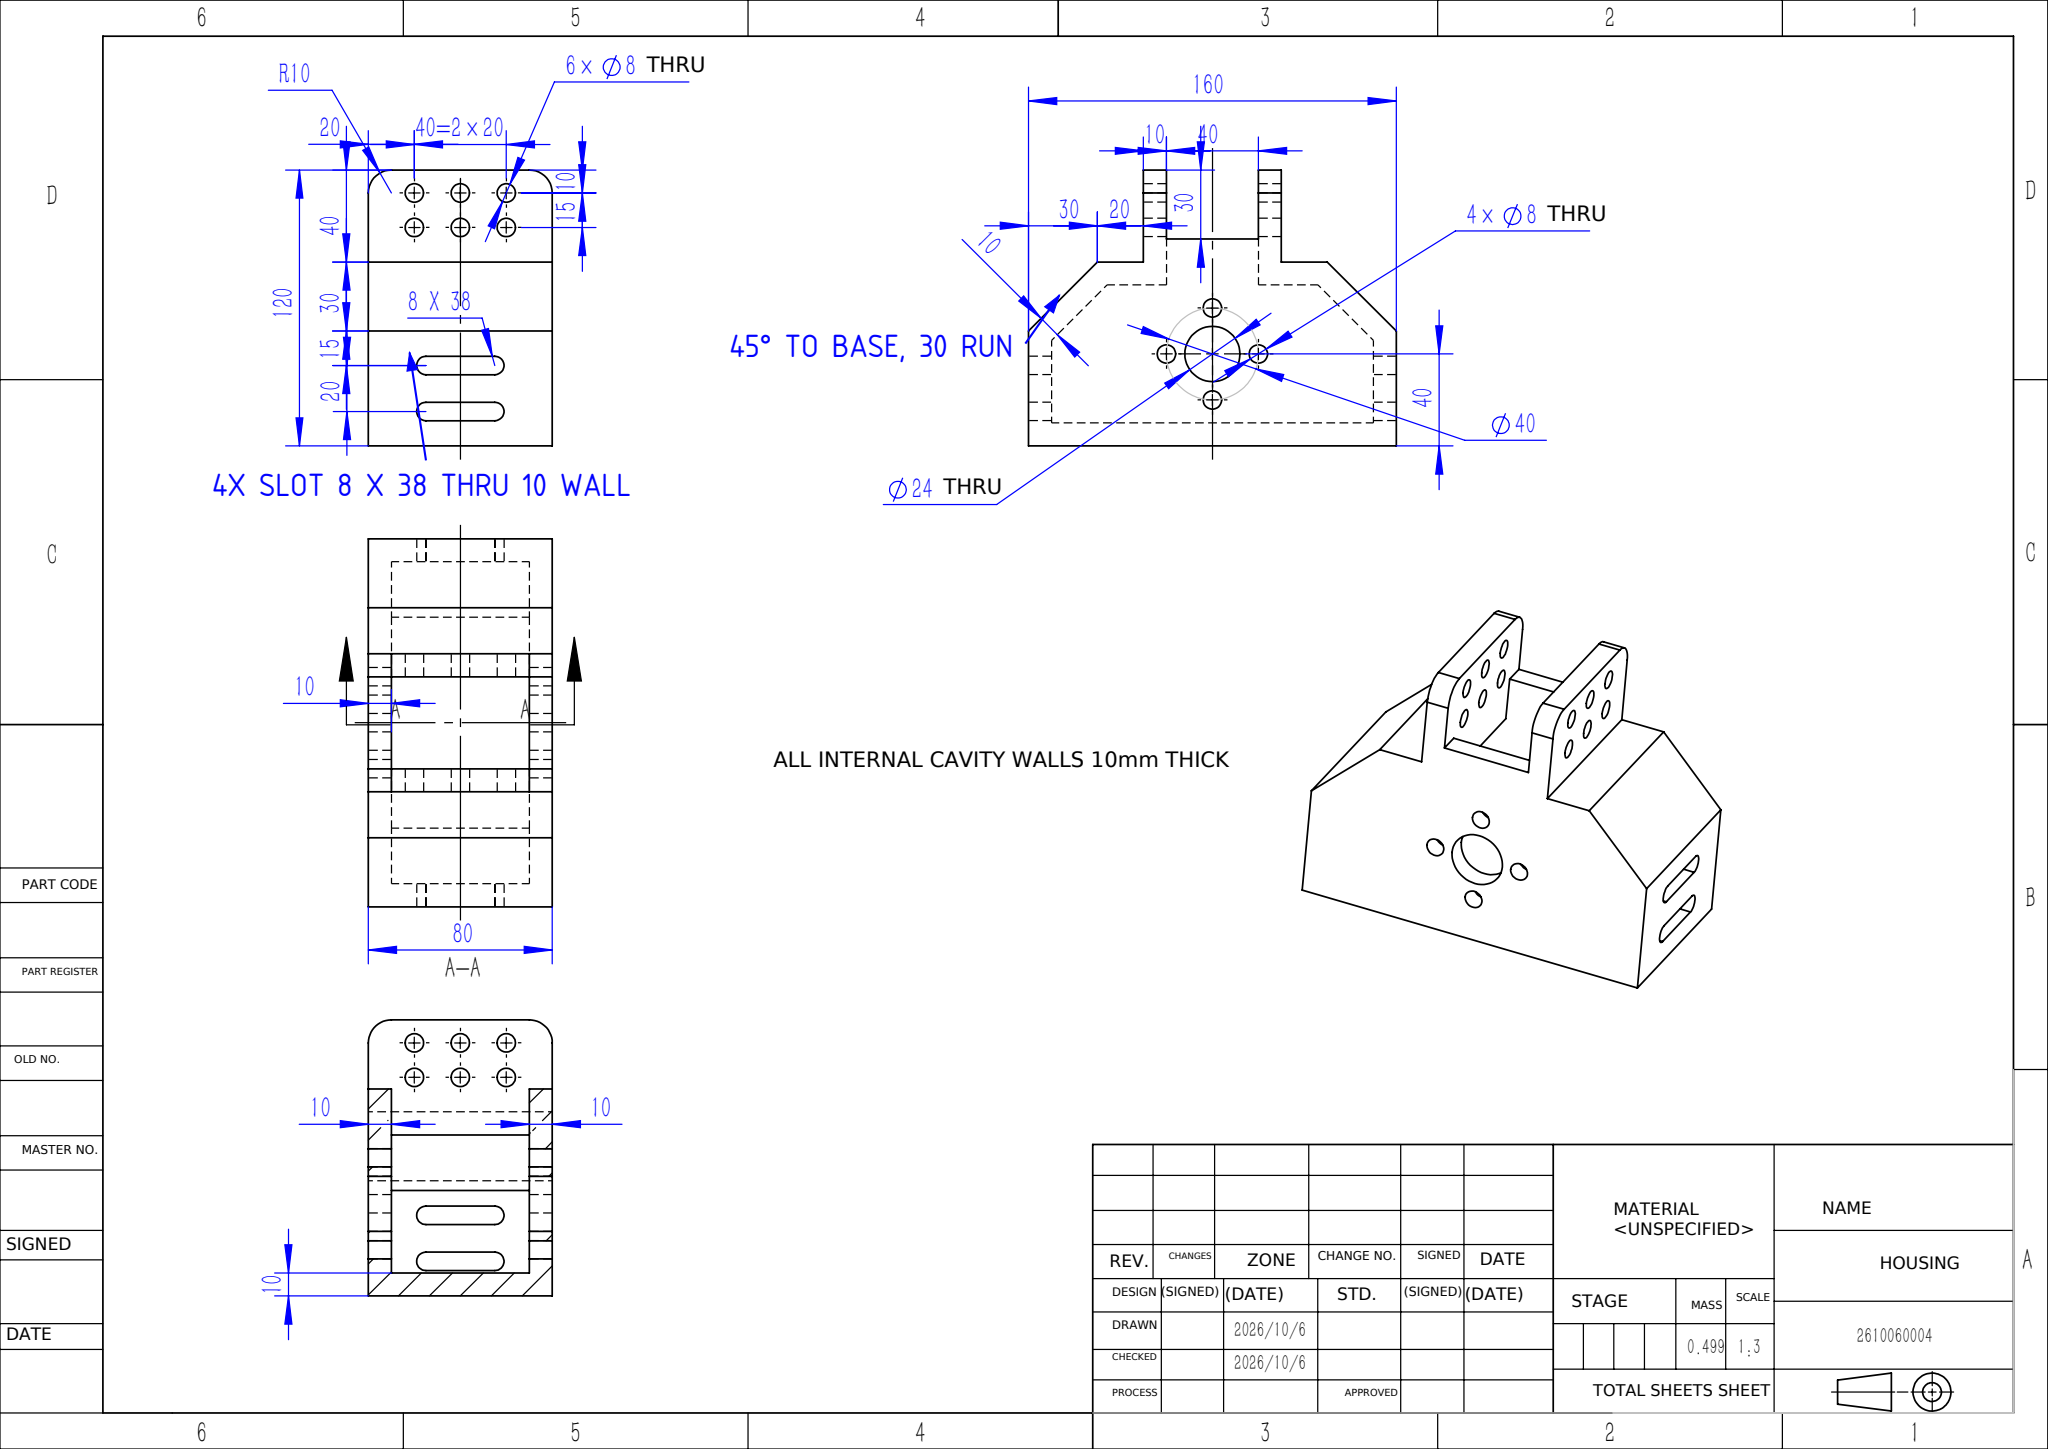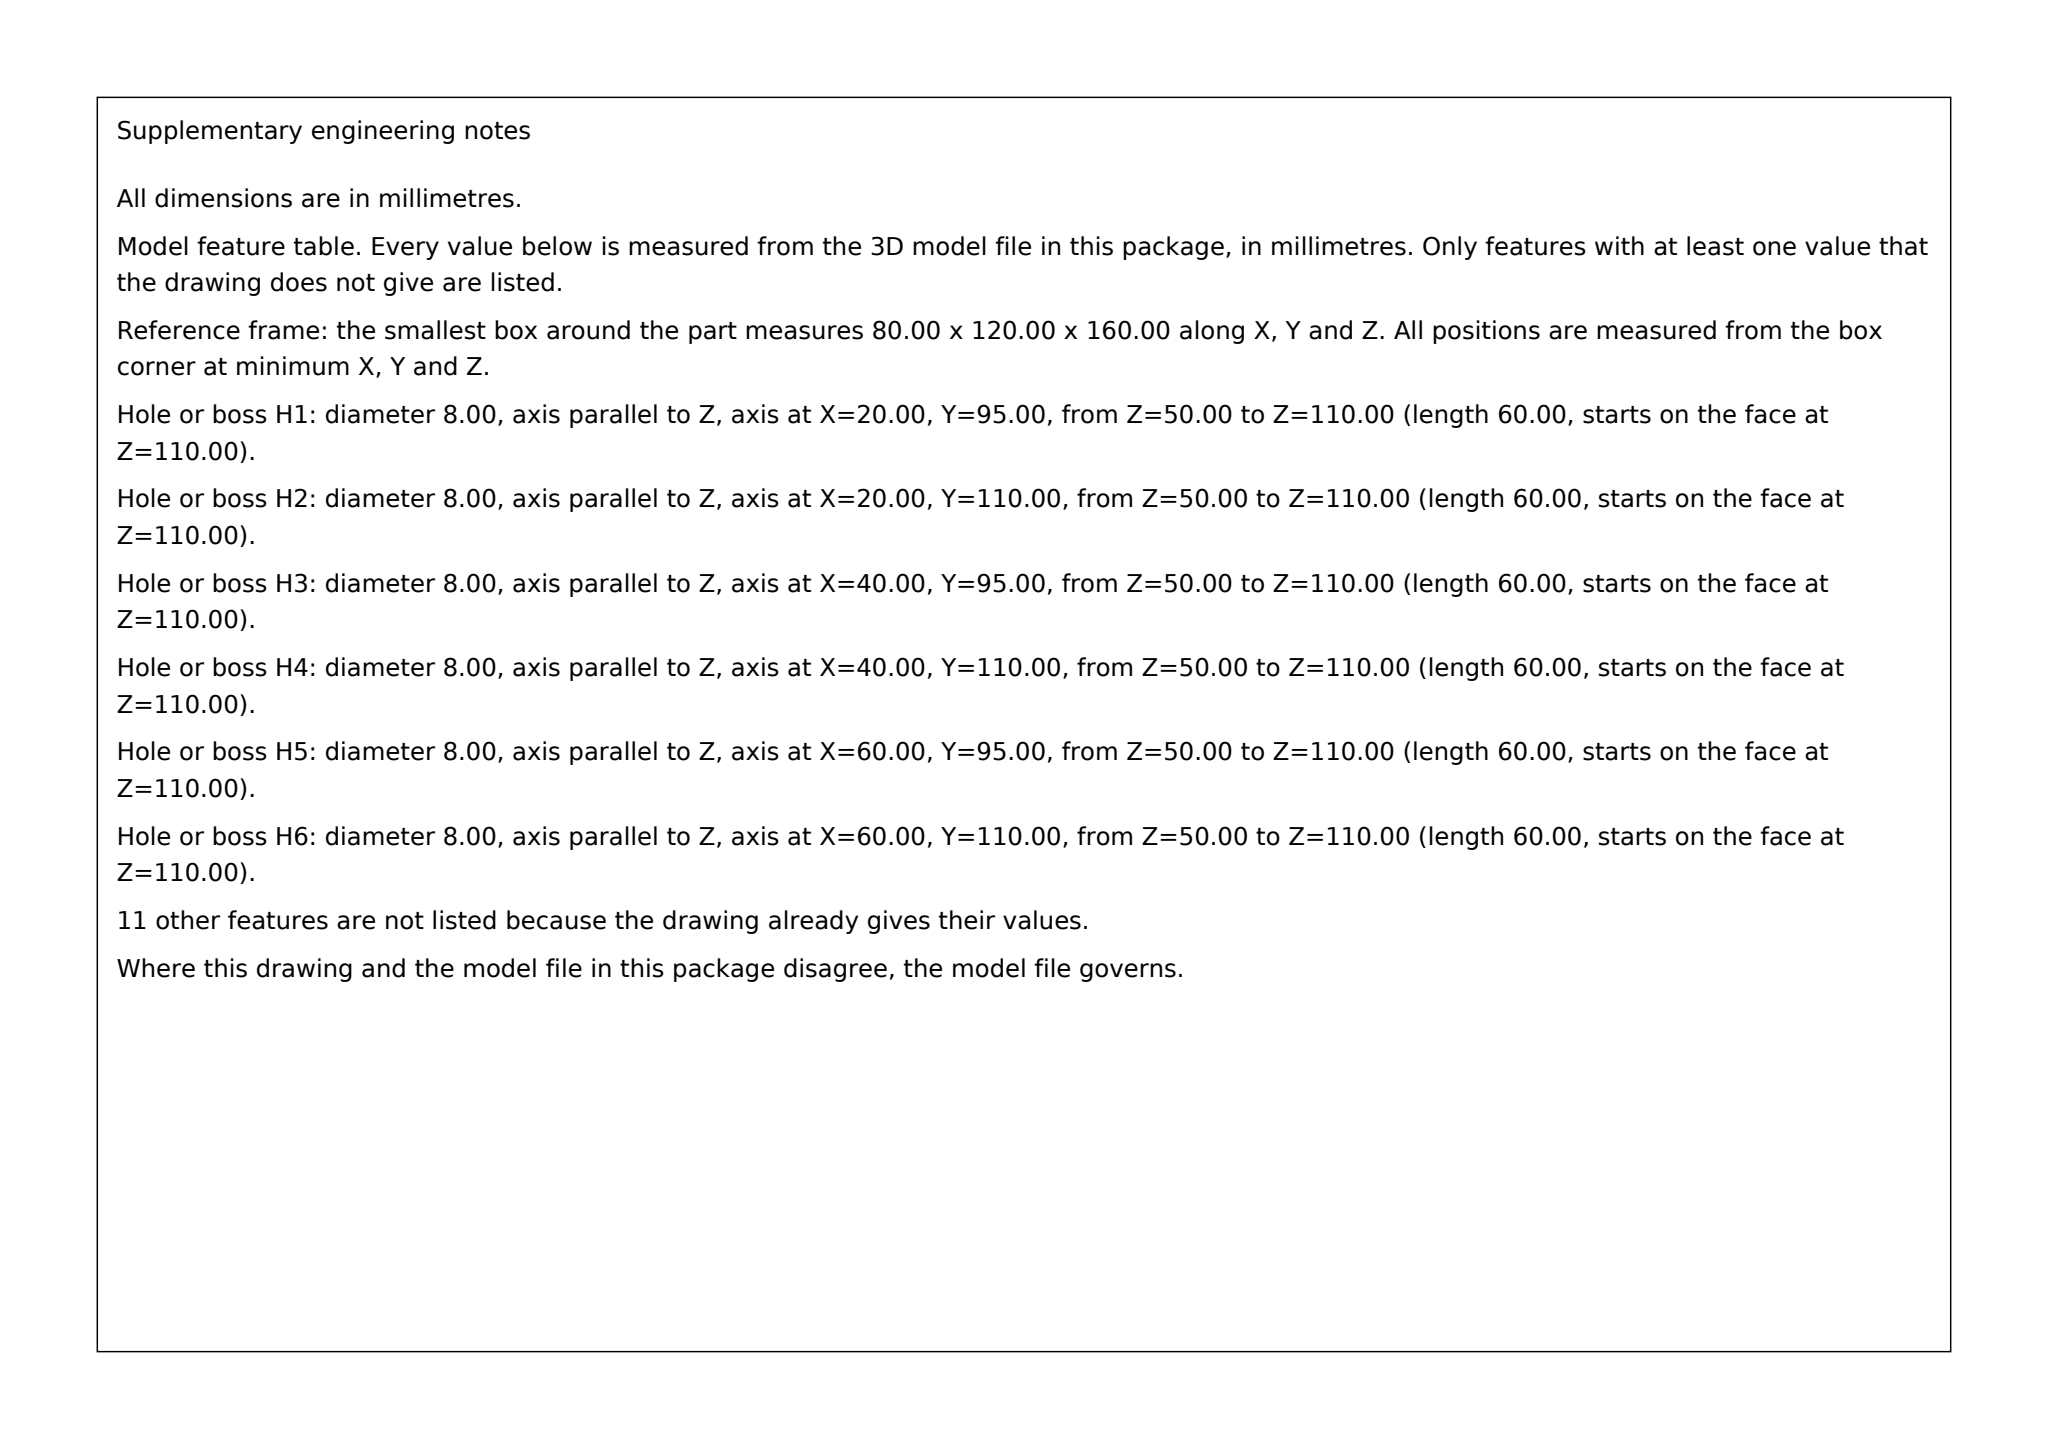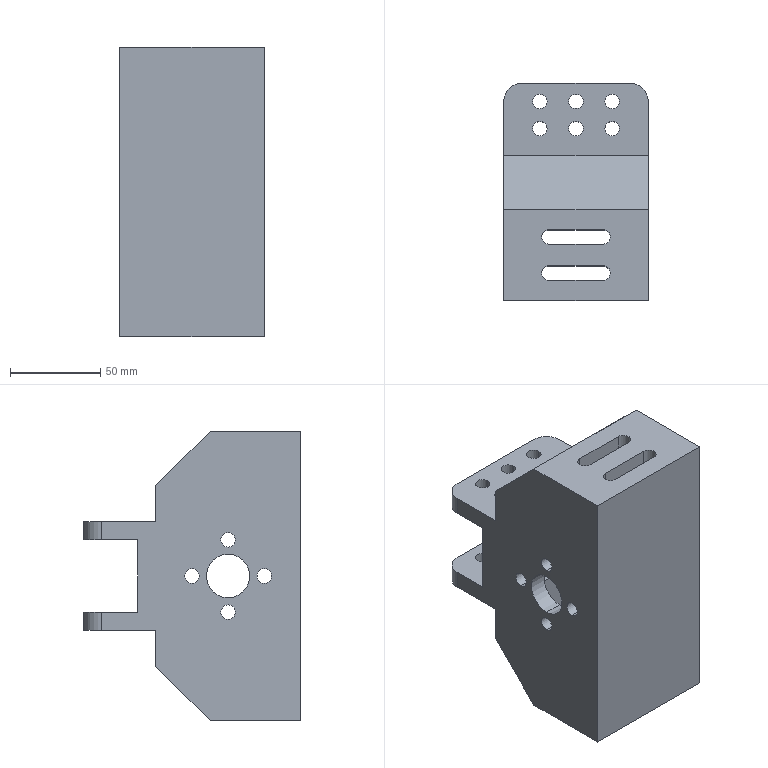Part | SolidWorks | mm | 1 solid | 94 faces | box 80 x 120 x 160 mm | volume 499401 mm3 | cylinder 60 | plane 34 | commonest cylinder face diameters 8 x52 24 x4 20 x4
Drawing notes:
INCL SIDE FACES 45° TO BASE: 30 RUN, 40 HIGH SIDE UP TO 70 HIGH TOP | from the solid: Front view (z-y) outline: vertical sides at z=0/z=160 end at y=40 (= Ø40 BC axis height, dim 40); top face plane y=70; slant horiz run 30 (dim 30) => rise 70-40=30, angle 45°. Cavity face parallel, offset 10.
SLOTS 8 WIDE X 38 LONG (END RADII R4 ON CENTERS X=25 AND X=55 FROM LEFT FACE) ARE THRU THE 10 THICK WALL; 2 PER WALL AT Y=15 AND Y=35 FROM BASE, IN BOTH END WALLS (Z=0-10 AND Z=150-160), 4 PLACES TOTAL | from the solid: cylinders: concave arc dia 8.0 axis z at [25,15],[55,15],[25,35],[55,35], from 0.0 to 10.0 and from 150.0 to 160.0; axis_planes y=11/19/31/39 extent x[25,55] z[0,10] and z[150,160]
build123d program:
from build123d import *

# Parameters (mm, degrees)
BOSS_EXTRUDE1_DEPTH = 40
CUT_EXTRUDE1_DEPTH  = 30
SKETCH3_W           = 80
SKETCH3_H           = 40
CUT_EXTRUDE2_DEPTH  = 30
SKETCH4_R           = 12
SKETCH4_R_2         = 4
CUT_EXTRUDE3_DEPTH  = 165.924
FILLET1_R           = 10
CUT_EXTRUDE4_DEPTH  = 204.961
SKETCH6_R           = 4
CUT_EXTRUDE5_DEPTH  = 168.631


with BuildPart() as part:
    # Sketch1 → Boss-Extrude1 (new, symmetric)
    with BuildSketch(Plane(origin=(0, 0, 0), x_dir=(0, 0, -1), z_dir=(1, 0, 0))):
        Polygon((80, 0), (-80, 0), (-80, 50), (-50, 80), (-30, 80), (-30, 120), (30, 120), (30, 80), (50, 80), (80, 50), align=None)
    extrude(amount=BOSS_EXTRUDE1_DEPTH, both=True)

    # Sketch2 → Cut-Extrude1 (cut, symmetric)
    with BuildSketch(Plane(origin=(0, 0, 0), x_dir=(0, 0, -1), z_dir=(1, 0, 0))):
        Polygon((20, 70), (20, 110), (-20, 110), (-20, 70), (-45.858, 70), (-70, 45.858), (-70, 10), (70, 10), (70, 45.858), (45.858, 70), align=None)
    extrude(amount=CUT_EXTRUDE1_DEPTH, both=True, mode=Mode.SUBTRACT)

    # Sketch3 → Cut-Extrude2 (cut)
    with BuildSketch(Plane(origin=(0, 120, 0), x_dir=(1, 0, 0), z_dir=(0, 1, 0))):
        Rectangle(SKETCH3_W, SKETCH3_H)
    extrude(amount=-CUT_EXTRUDE2_DEPTH, mode=Mode.SUBTRACT)

    # Sketch4 → Cut-Extrude3 (cut, through all)
    with BuildSketch(Plane.ZY.offset(40)):
        with Locations((0, 40)):
            Circle(SKETCH4_R)
        with Locations((0, 60)):
            Circle(SKETCH4_R_2)
        with Locations((20, 40)):
            Circle(SKETCH4_R_2)
        with Locations((0, 20)):
            Circle(SKETCH4_R_2)
        with Locations((-20, 40)):
            Circle(SKETCH4_R_2)
    extrude(amount=-CUT_EXTRUDE3_DEPTH, mode=Mode.SUBTRACT)

    # Fillet1
    fillet1_edges = [part.edges().sort_by_distance(p)[0] for p in [
        (-40, 120, -25),
        (40, 120, -25),
        (-40, 120, 25),
        (40, 120, 25),
    ]]
    fillet(fillet1_edges, radius=FILLET1_R)

    # Sketch5 → Cut-Extrude4 (cut, through all)
    with BuildSketch(Plane(origin=(0, 0, -80), x_dir=(-1, 0, 0), z_dir=(0, 0, -1))):
        with BuildLine():
            Line((-15, 39), (15, 39))
            ThreePointArc((15, 39), (19, 35), (15, 31))
            Line((15, 31), (-15, 31))
            ThreePointArc((-15, 31), (-19, 35), (-15, 39))
        make_face()
        with BuildLine():
            Line((-15, 19), (15, 19))
            ThreePointArc((15, 19), (19, 15), (15, 11))
            Line((15, 11), (-15, 11))
            ThreePointArc((-15, 11), (-19, 15), (-15, 19))
        make_face()
    extrude(amount=-CUT_EXTRUDE4_DEPTH, mode=Mode.SUBTRACT)

    # Sketch6 → Cut-Extrude5 (cut, through all)
    with BuildSketch(Plane.XY.offset(30)):
        with Locations((-20, 110)):
            Circle(SKETCH6_R)
        with Locations((0, 110)):
            Circle(SKETCH6_R)
        with Locations((20, 110)):
            Circle(SKETCH6_R)
        with Locations((-20, 95)):
            Circle(SKETCH6_R)
        with Locations((0, 95)):
            Circle(SKETCH6_R)
        with Locations((20, 95)):
            Circle(SKETCH6_R)
    extrude(amount=-CUT_EXTRUDE5_DEPTH, mode=Mode.SUBTRACT)


solid = part.part